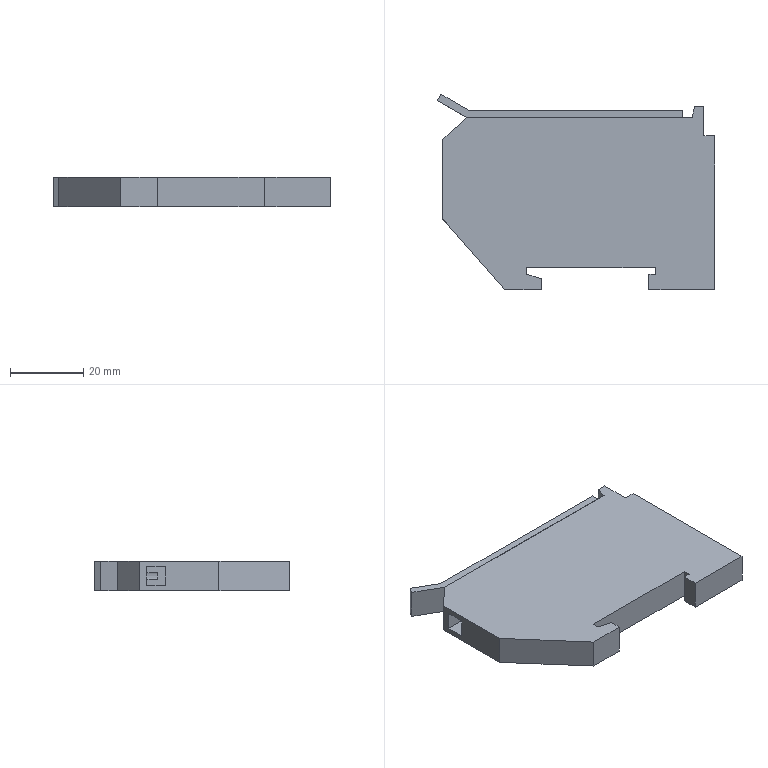Component | SolidWorks | UK5NFuseTerminal-1 | 2 solids | 58 faces | volume 24981 mm3 | plane 49 | cylinder 9 | commonest cylinder face diameters 5 x9